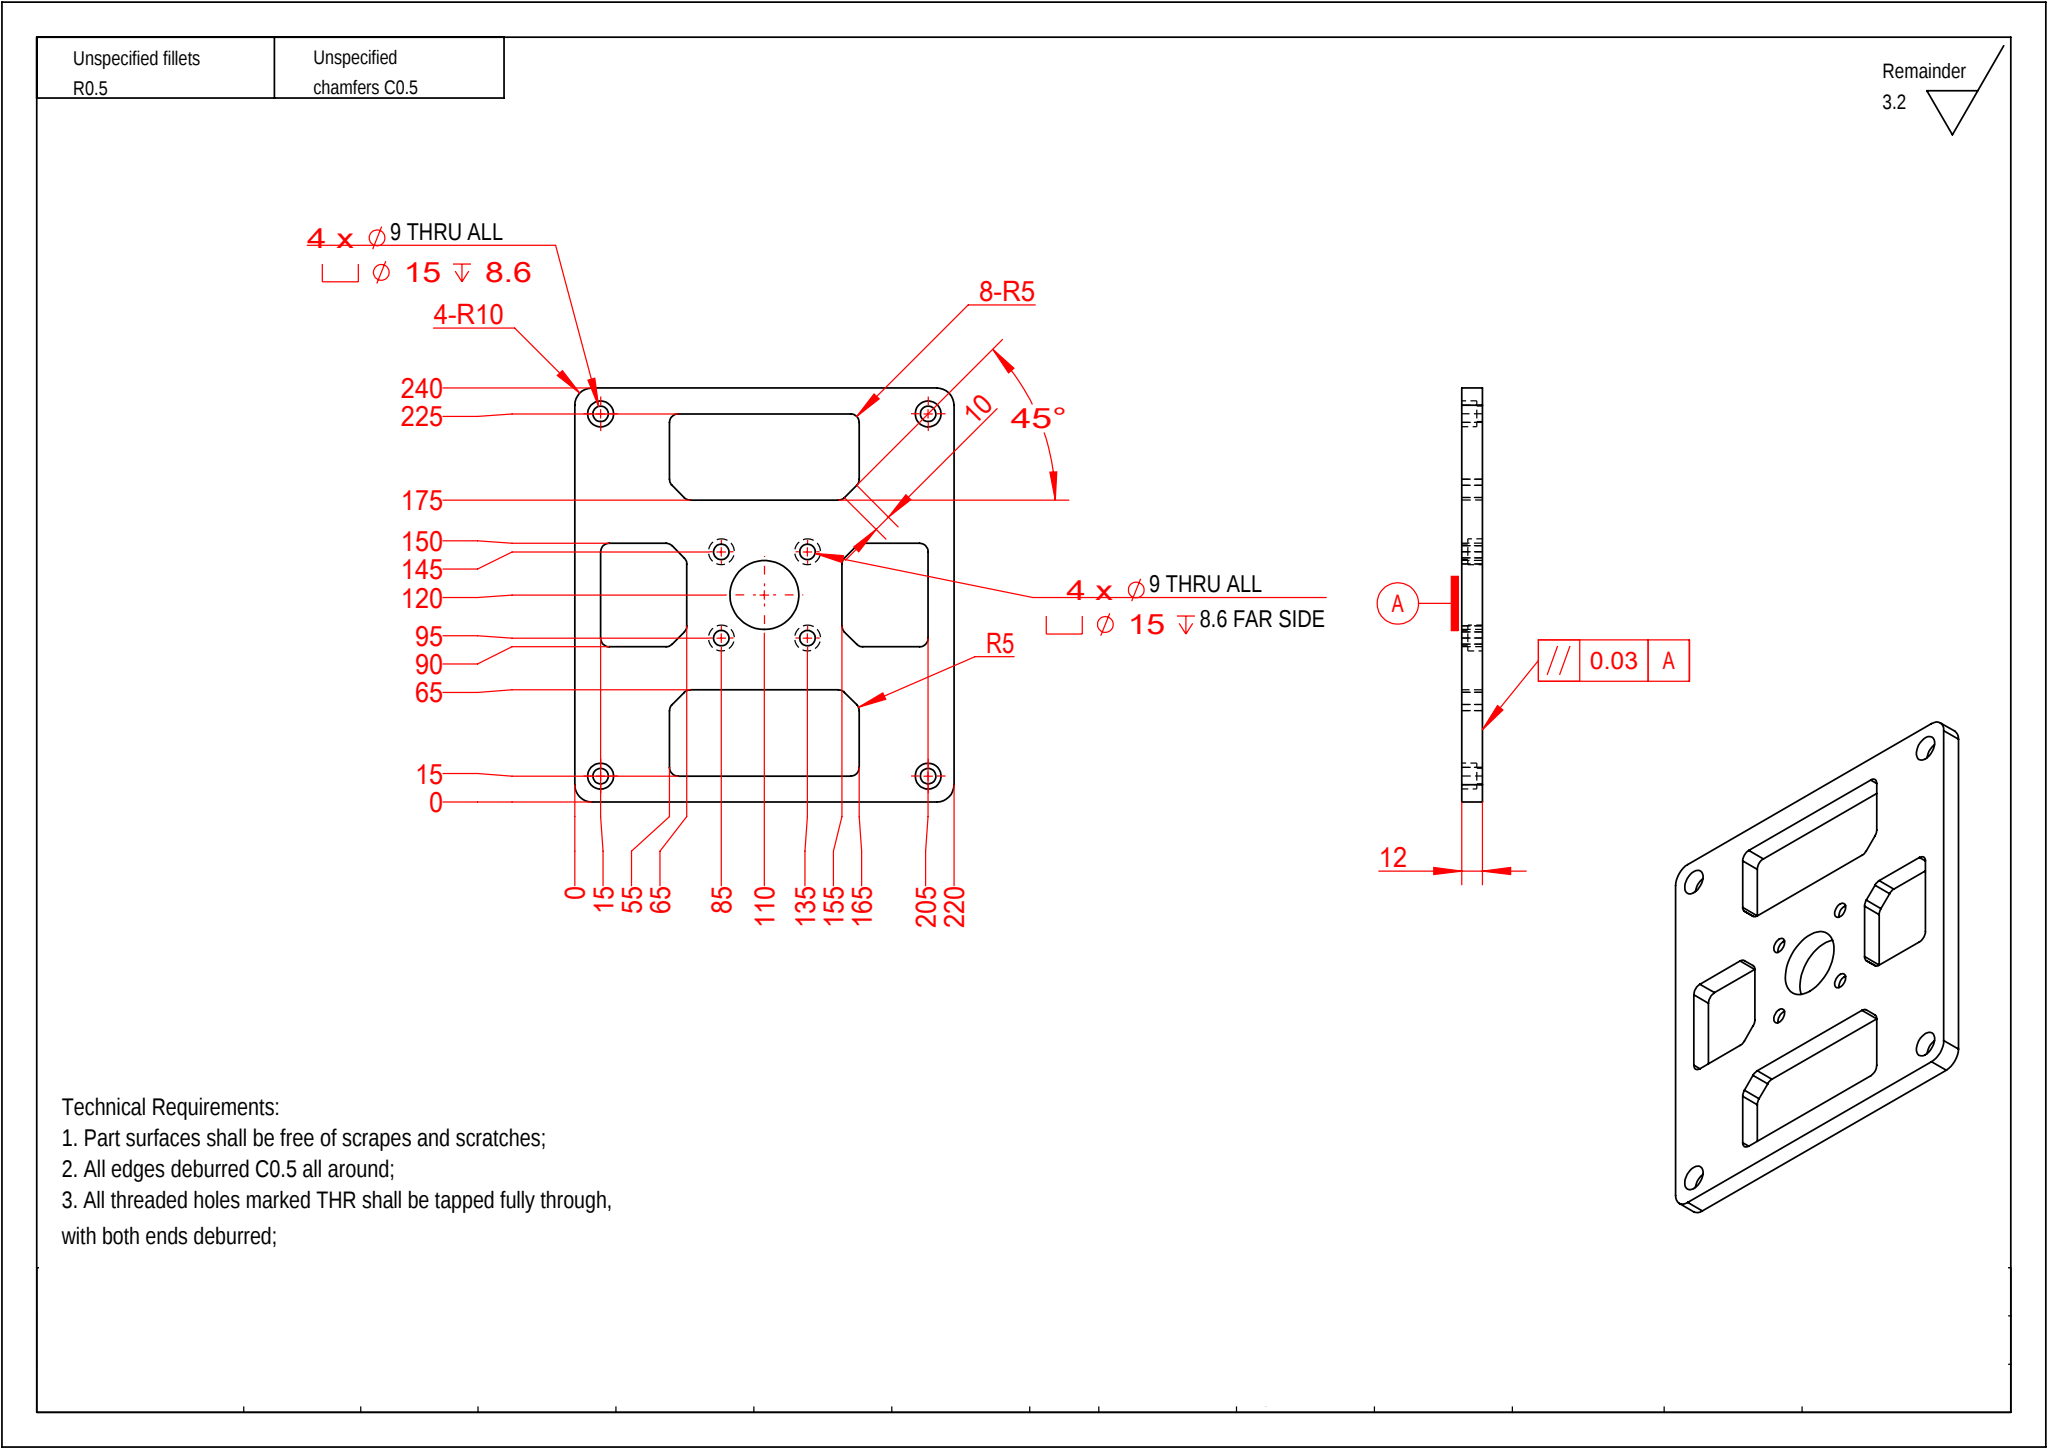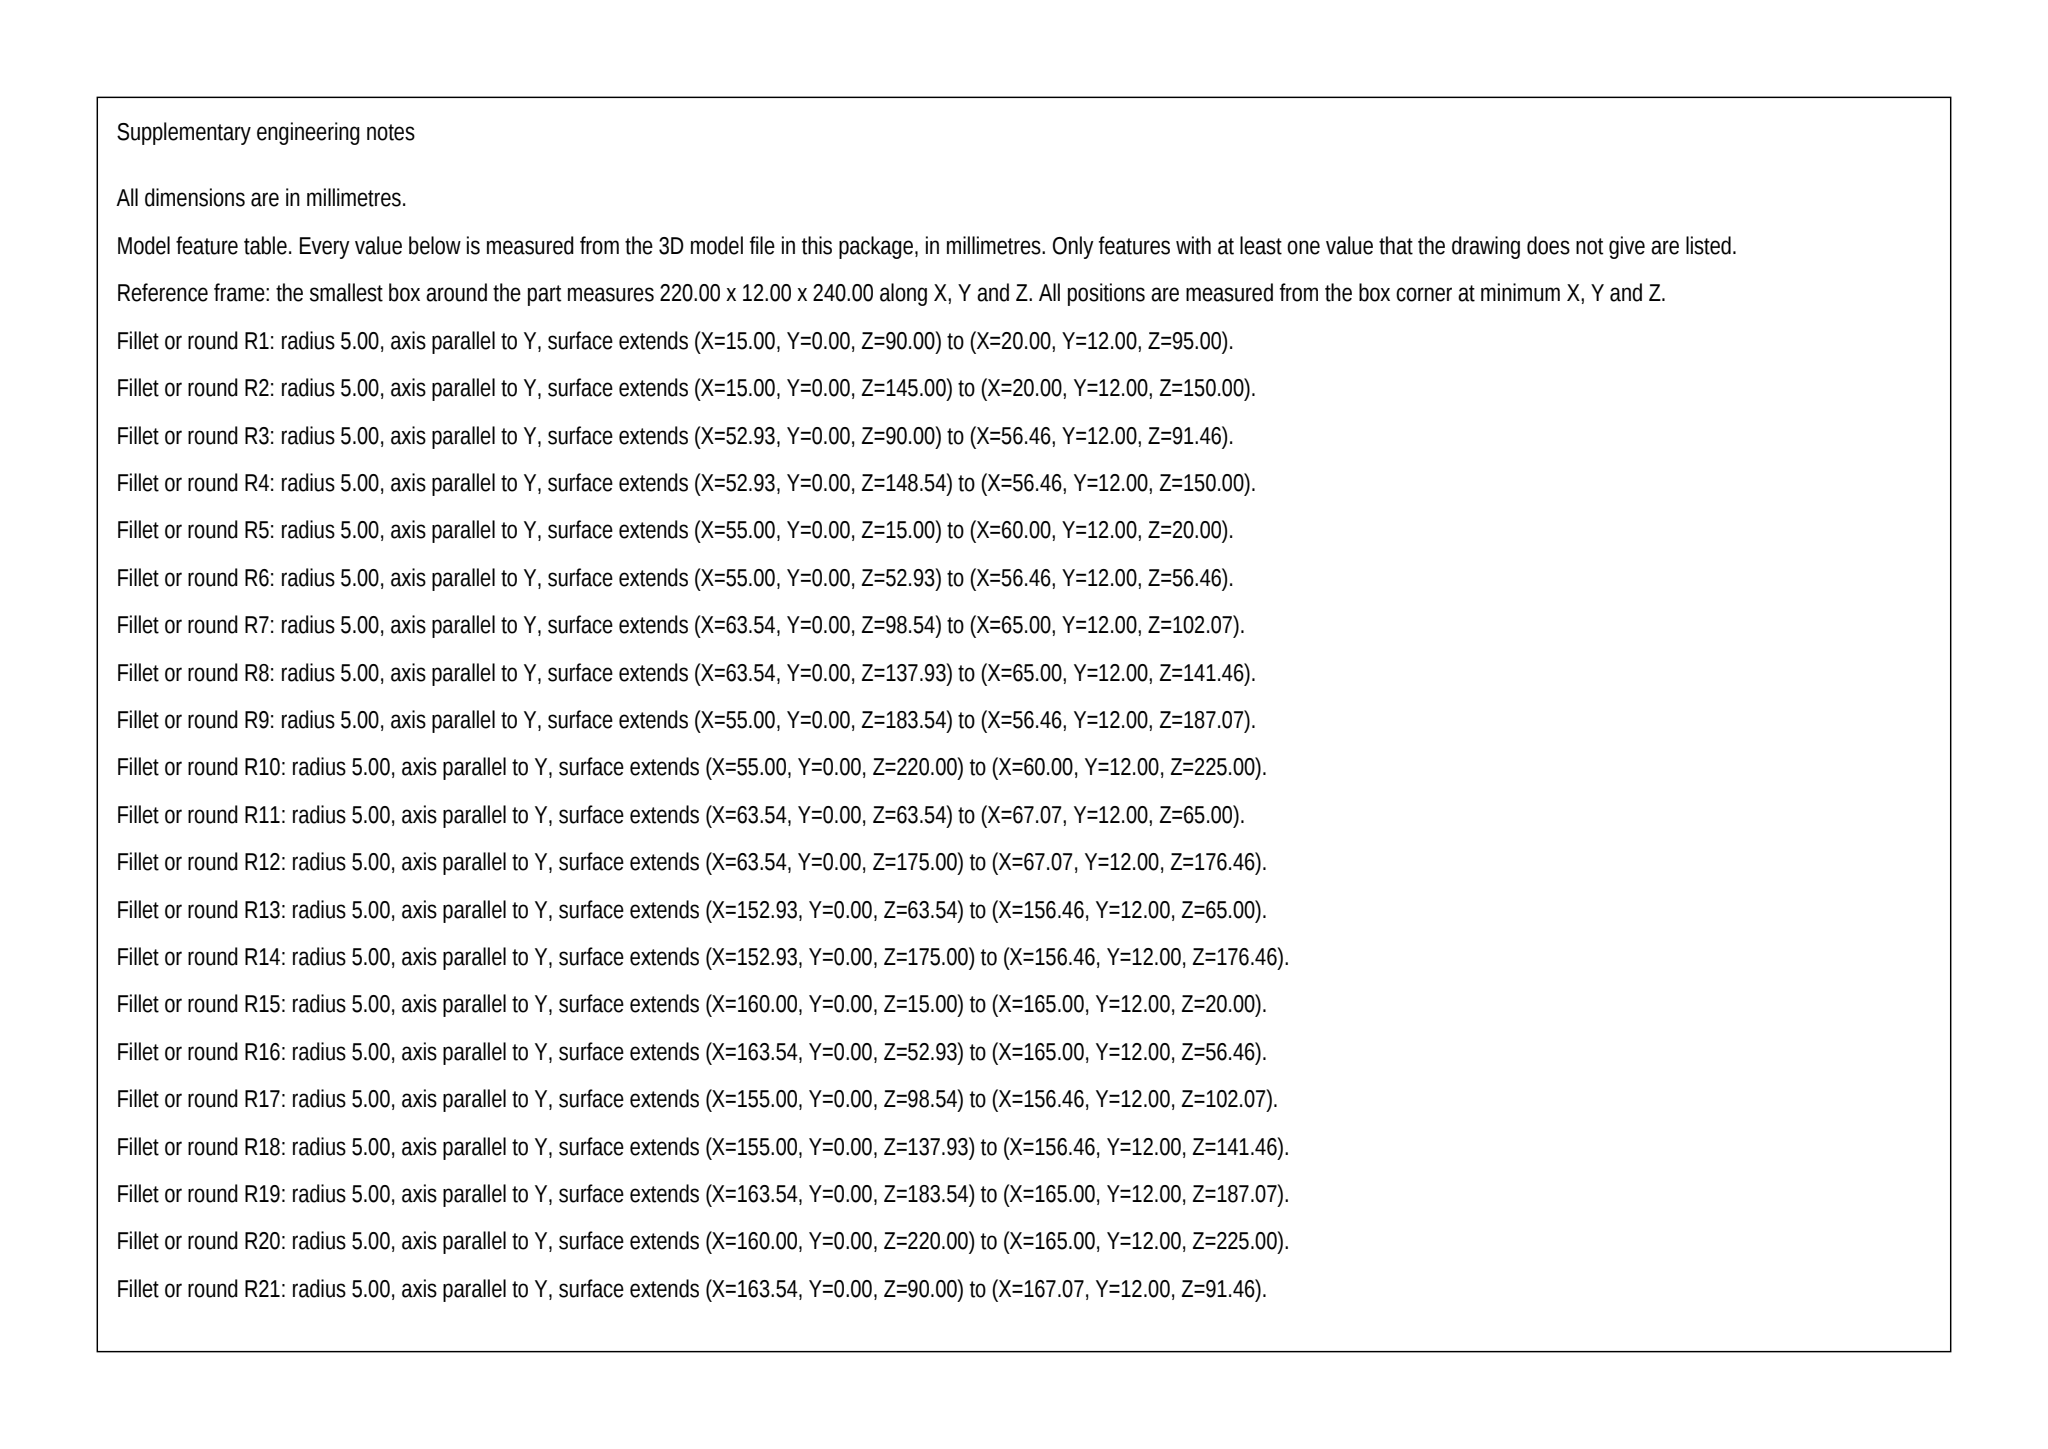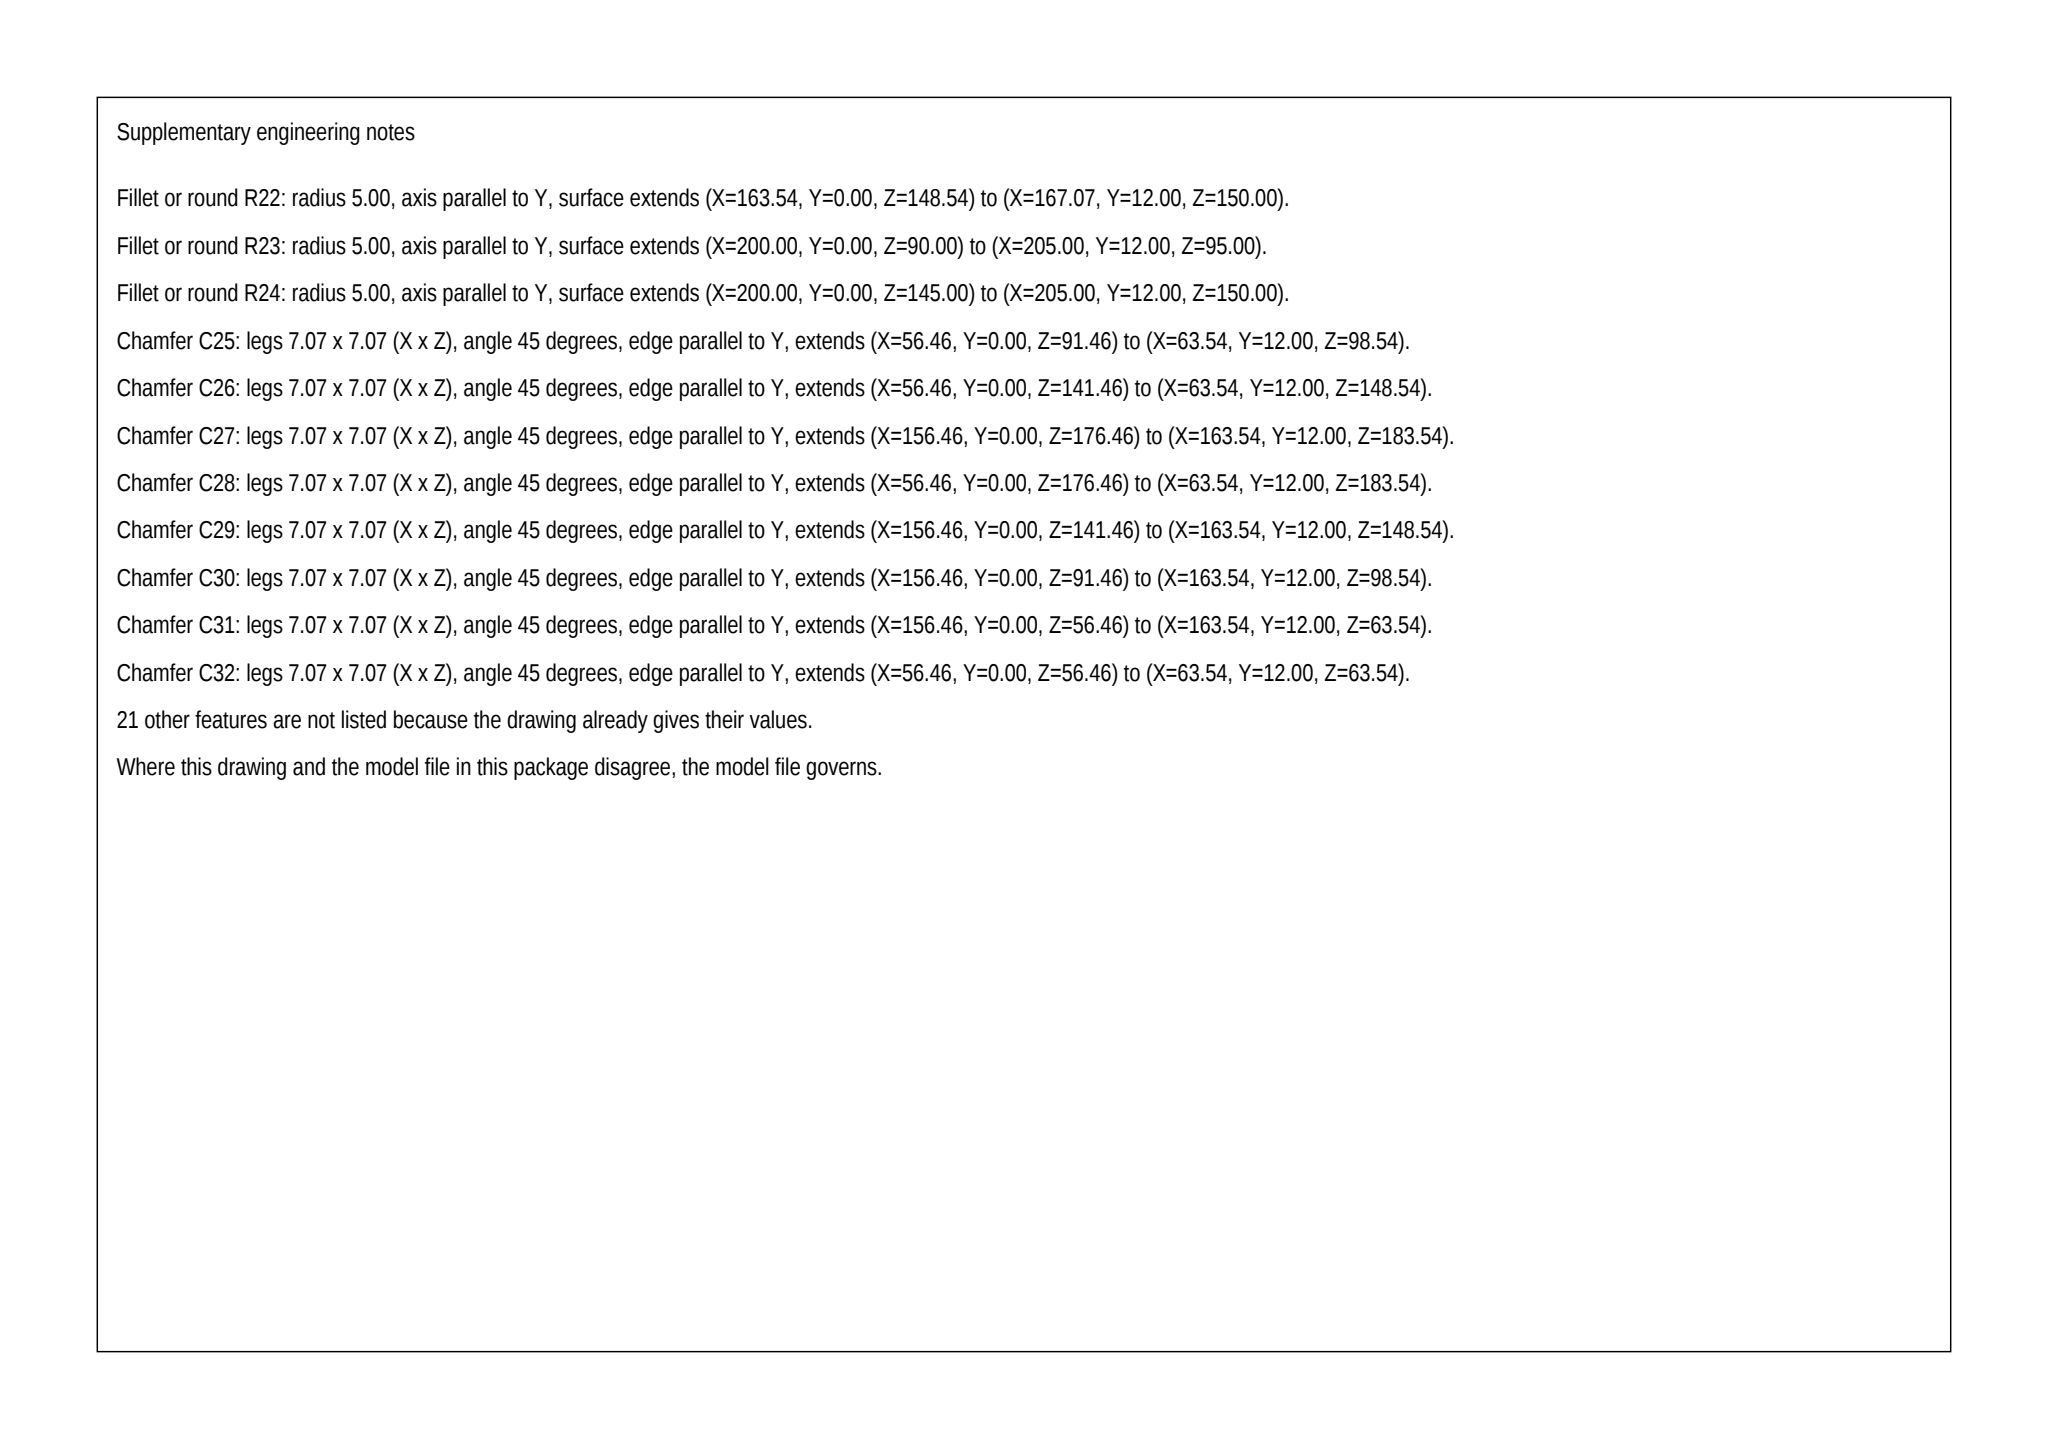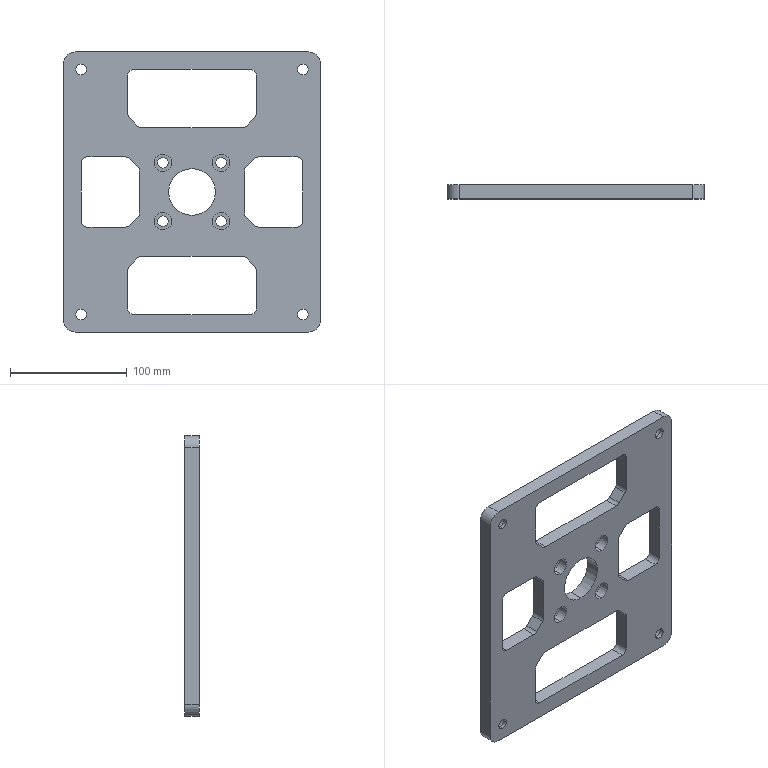Part | SolidWorks | mm | 1 solid | 100 faces | box 220 x 12 x 240 mm | volume 405020 mm3 | cylinder 62 | plane 38 | commonest cylinder face diameters 10 x24 15 x16 9 x16 20 x4 40 x2
build123d program:
from build123d import *

# Parameters (mm, degrees)
SKETCH1_W                                       = 220
SKETCH1_H                                       = 240
BOSS_EXTRUDE1_DEPTH                             = 12
FILLET1_R                                       = 10
M8_HEX_SOCKET_HEAD_CAP_SCREW_CBORE1_D           = 9
M8_HEX_SOCKET_HEAD_CAP_SCREW_CBORE1_CBORE_D     = 15
M8_HEX_SOCKET_HEAD_CAP_SCREW_CBORE1_CBORE_DEPTH = 8.6
SKETCH5_R                                       = 20
CUT_EXTRUDE1_DEPTH                              = 32.655
M8_HEX_SOCKET_HEAD_CAP_SCREW_CBORE2_D           = 9
M8_HEX_SOCKET_HEAD_CAP_SCREW_CBORE2_CBORE_D     = 15
M8_HEX_SOCKET_HEAD_CAP_SCREW_CBORE2_CBORE_DEPTH = 8.6
SKETCH8_W                                       = 110
SKETCH8_H                                       = 50
SKETCH8_W_2                                     = 50
SKETCH8_H_2                                     = 60
CUT_EXTRUDE2_DEPTH                              = 164.23
CHAMFER1_SIZE                                   = 10
FILLET2_R                                       = 5


with BuildPart() as part:
    # Sketch1 → Boss-Extrude1 (new body)
    with BuildSketch(Plane(origin=(0, 0, 0), x_dir=(1, 0, 0), z_dir=(0, 1, 0))):
        Rectangle(SKETCH1_W, SKETCH1_H)
    extrude(amount=BOSS_EXTRUDE1_DEPTH)

    # Fillet1
    fillet1_edges = [part.edges().sort_by_distance(p)[0] for p in [
        (110, 6, 120),
        (-110, 6, 120),
        (-110, 6, -120),
        (110, 6, -120),
    ]]
    fillet(fillet1_edges, radius=FILLET1_R)

    # M8 Hex Socket Head Cap Screw CBORE1 (through all)
    with Locations(Plane(origin=(0, 12, 0), x_dir=(1, 0, 0), z_dir=(0, 1, 0))):
        with Locations((-95, 105), (95, 105), (-95, -105), (95, -105)):
            CounterBoreHole(M8_HEX_SOCKET_HEAD_CAP_SCREW_CBORE1_D / 2, M8_HEX_SOCKET_HEAD_CAP_SCREW_CBORE1_CBORE_D / 2, M8_HEX_SOCKET_HEAD_CAP_SCREW_CBORE1_CBORE_DEPTH)

    # Sketch5 → Cut-Extrude1 (cut)
    with BuildSketch(Plane(origin=(0, 12, 0), x_dir=(1, 0, 0), z_dir=(0, 1, 0))):
        with Locations(Location((0, 0, 0), (0, 0, 270))):
            Circle(SKETCH5_R)
    extrude(amount=-CUT_EXTRUDE1_DEPTH, mode=Mode.SUBTRACT)

    # M8 Hex Socket Head Cap Screw CBORE2 (through all)
    with Locations(Plane(origin=(0, 0, 0), x_dir=(-1, 0, 0), z_dir=(0, -1, 0))):
        with Locations((-25, -25), (25, -25), (25, 25), (-25, 25)):
            CounterBoreHole(M8_HEX_SOCKET_HEAD_CAP_SCREW_CBORE2_D / 2, M8_HEX_SOCKET_HEAD_CAP_SCREW_CBORE2_CBORE_D / 2, M8_HEX_SOCKET_HEAD_CAP_SCREW_CBORE2_CBORE_DEPTH)

    # Sketch8 → Cut-Extrude2 (cut, through all)
    with BuildSketch(Plane(origin=(0, 12, 0), x_dir=(1, 0, 0), z_dir=(0, 1, 0))):
        with Locations((0, 80)):
            Rectangle(SKETCH8_W, SKETCH8_H)
        with Locations((0, -80)):
            Rectangle(SKETCH8_W, SKETCH8_H)
        with Locations((-70, 0)):
            Rectangle(SKETCH8_W_2, SKETCH8_H_2)
        with Locations((70, 0)):
            Rectangle(SKETCH8_W_2, SKETCH8_H_2)
    extrude(amount=-CUT_EXTRUDE2_DEPTH, mode=Mode.SUBTRACT)

    # Chamfer1
    chamfer1_edges = [part.edges().sort_by_distance(p)[0] for p in [
        (55, 6, -55),
        (-55, 6, -55),
        (-55, 6, 55),
        (55, 6, 55),
        (-45, 6, -30),
        (-45, 6, 30),
        (45, 6, 30),
        (45, 6, -30),
    ]]
    chamfer(chamfer1_edges, length=CHAMFER1_SIZE)

    # Fillet2
    fillet2_edges = [part.edges().sort_by_distance(p)[0] for p in [
        (55, 6, -105),
        (-55, 6, -105),
        (-55, 6, 105),
        (55, 6, 105),
        (-95, 6, 30),
        (-95, 6, -30),
        (95, 6, -30),
        (95, 6, 30),
        (-55, 6, -30),
        (-45, 6, 20),
        (-45, 6, -20),
        (-55, 6, 30),
        (-45, 6, 55),
        (45, 6, 55),
        (55, 6, 65),
        (-55, 6, 65),
        (55, 6, 30),
        (45, 6, -20),
        (45, 6, 20),
        (55, 6, -30),
        (55, 6, -65),
        (-45, 6, -55),
        (45, 6, -55),
        (-55, 6, -65),
    ]]
    fillet(fillet2_edges, radius=FILLET2_R)


solid = part.part